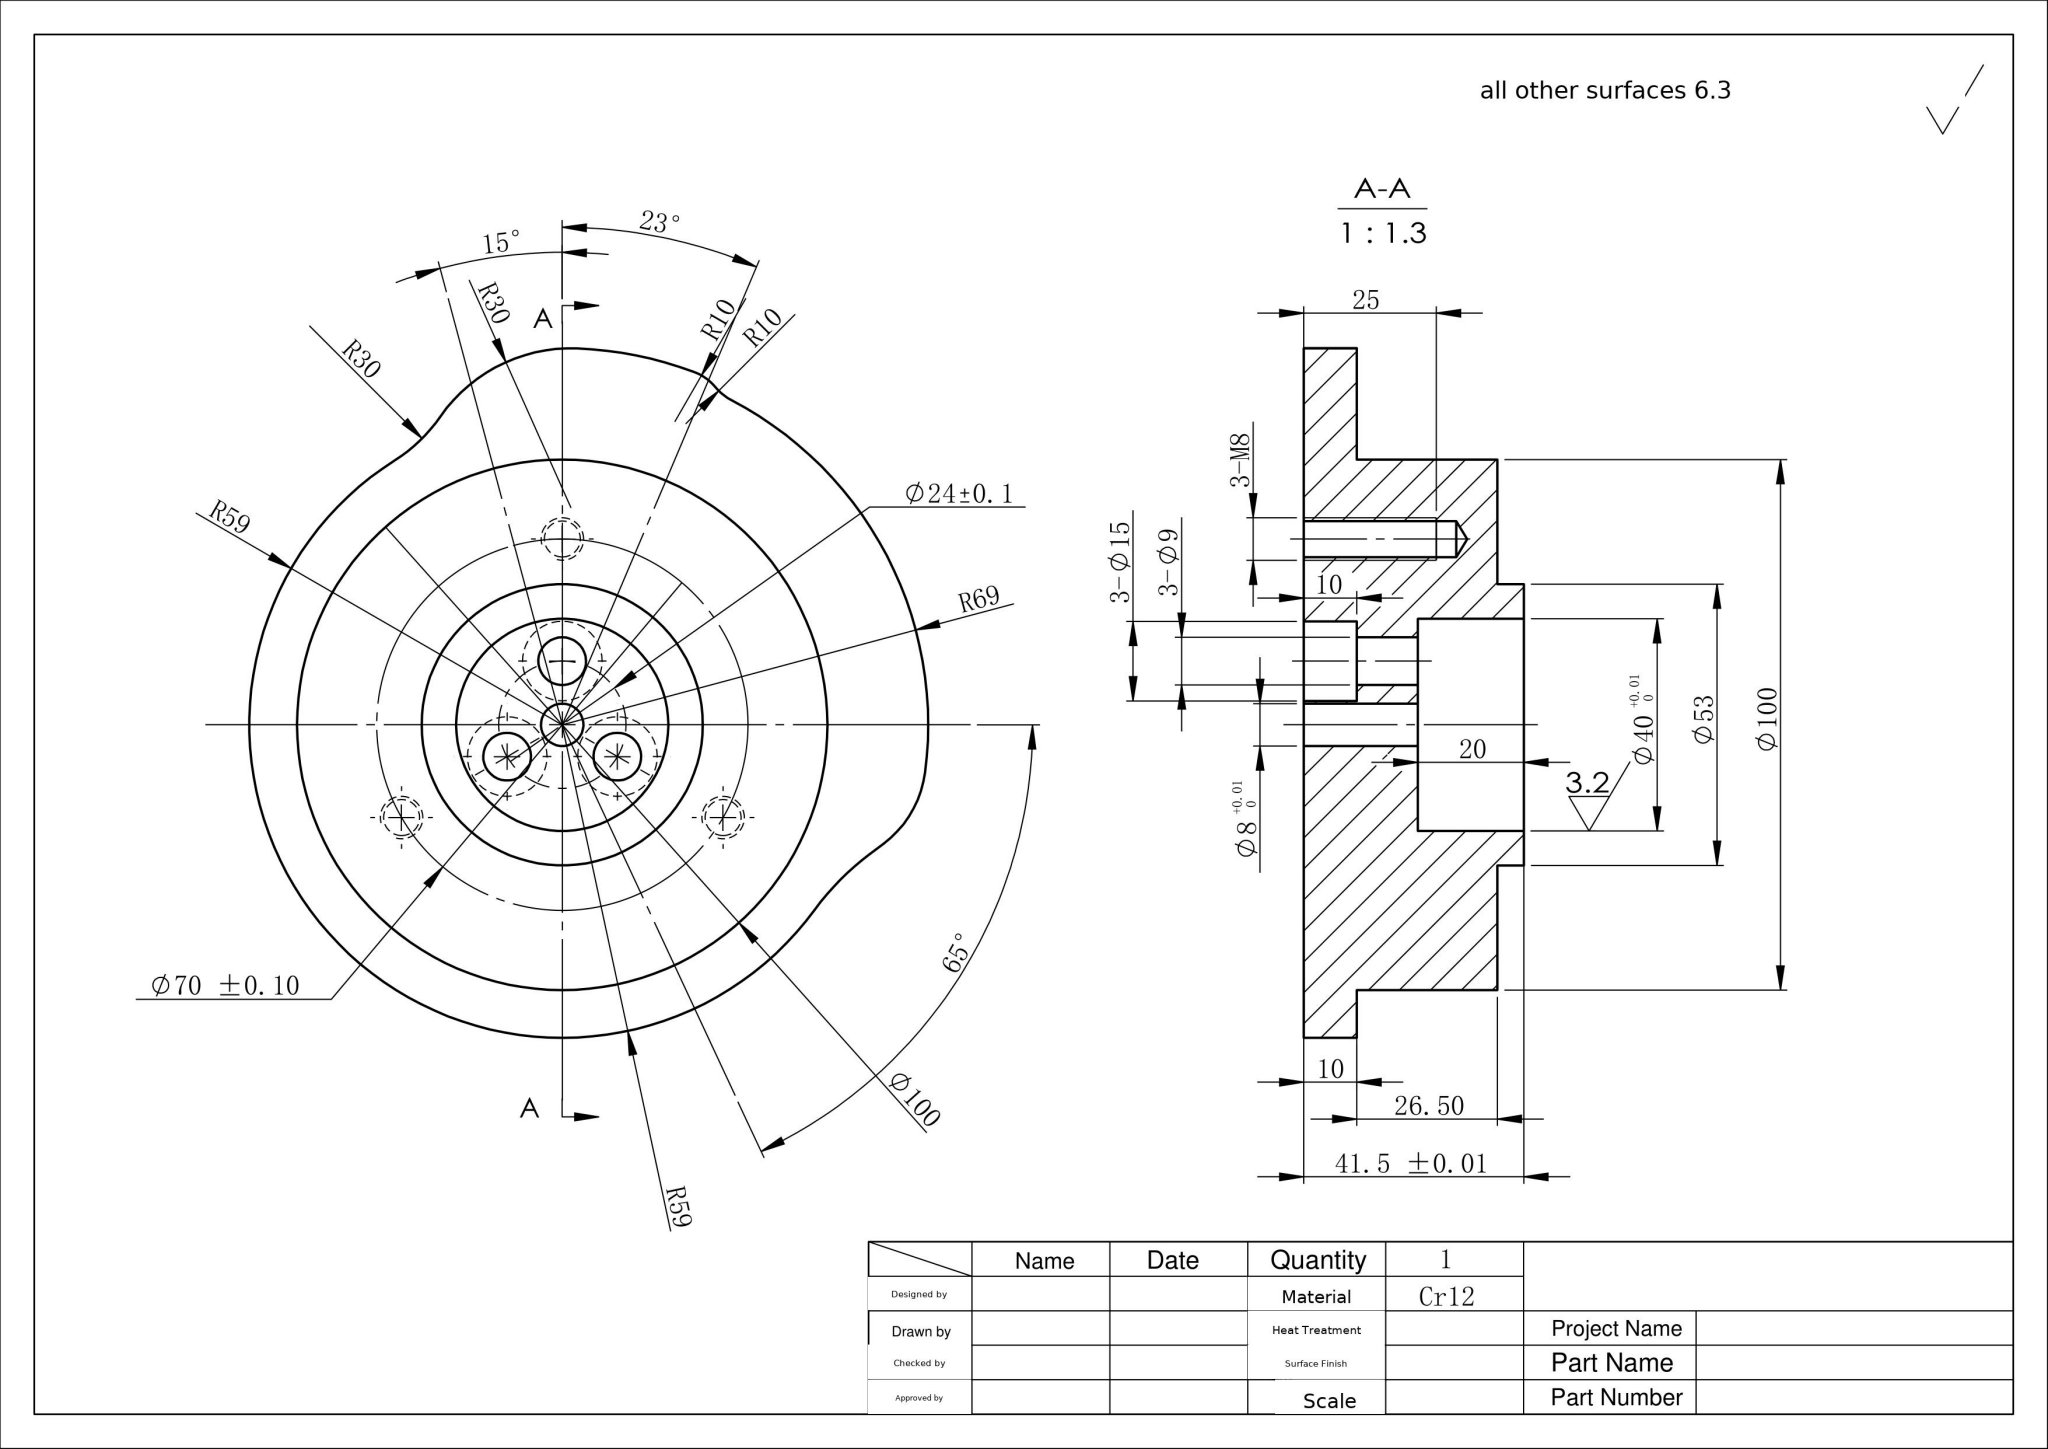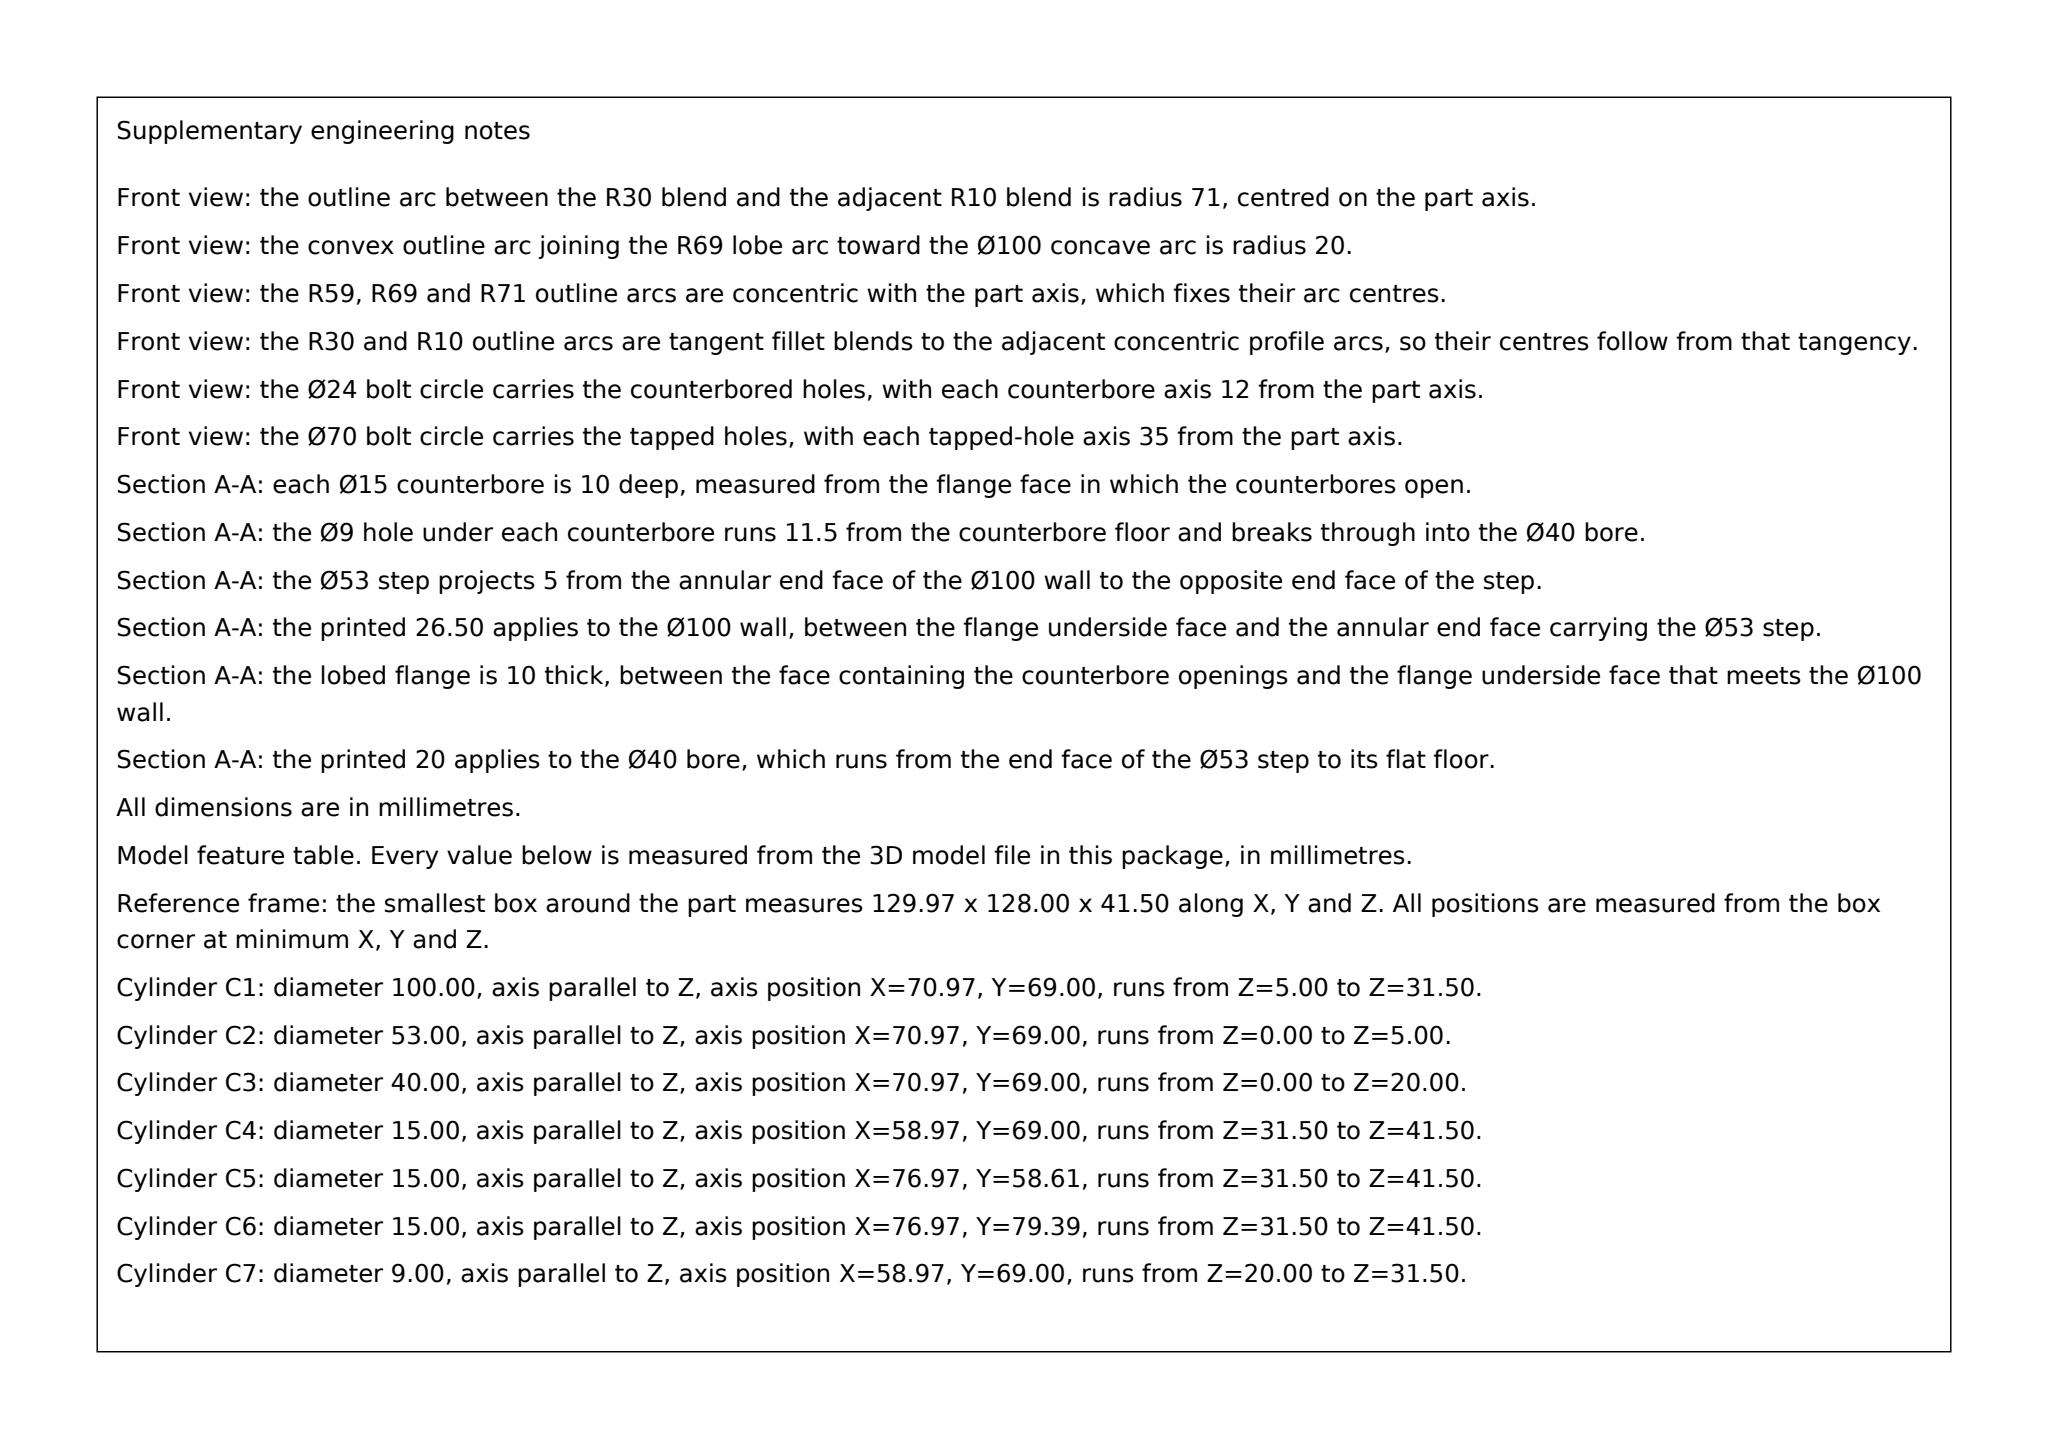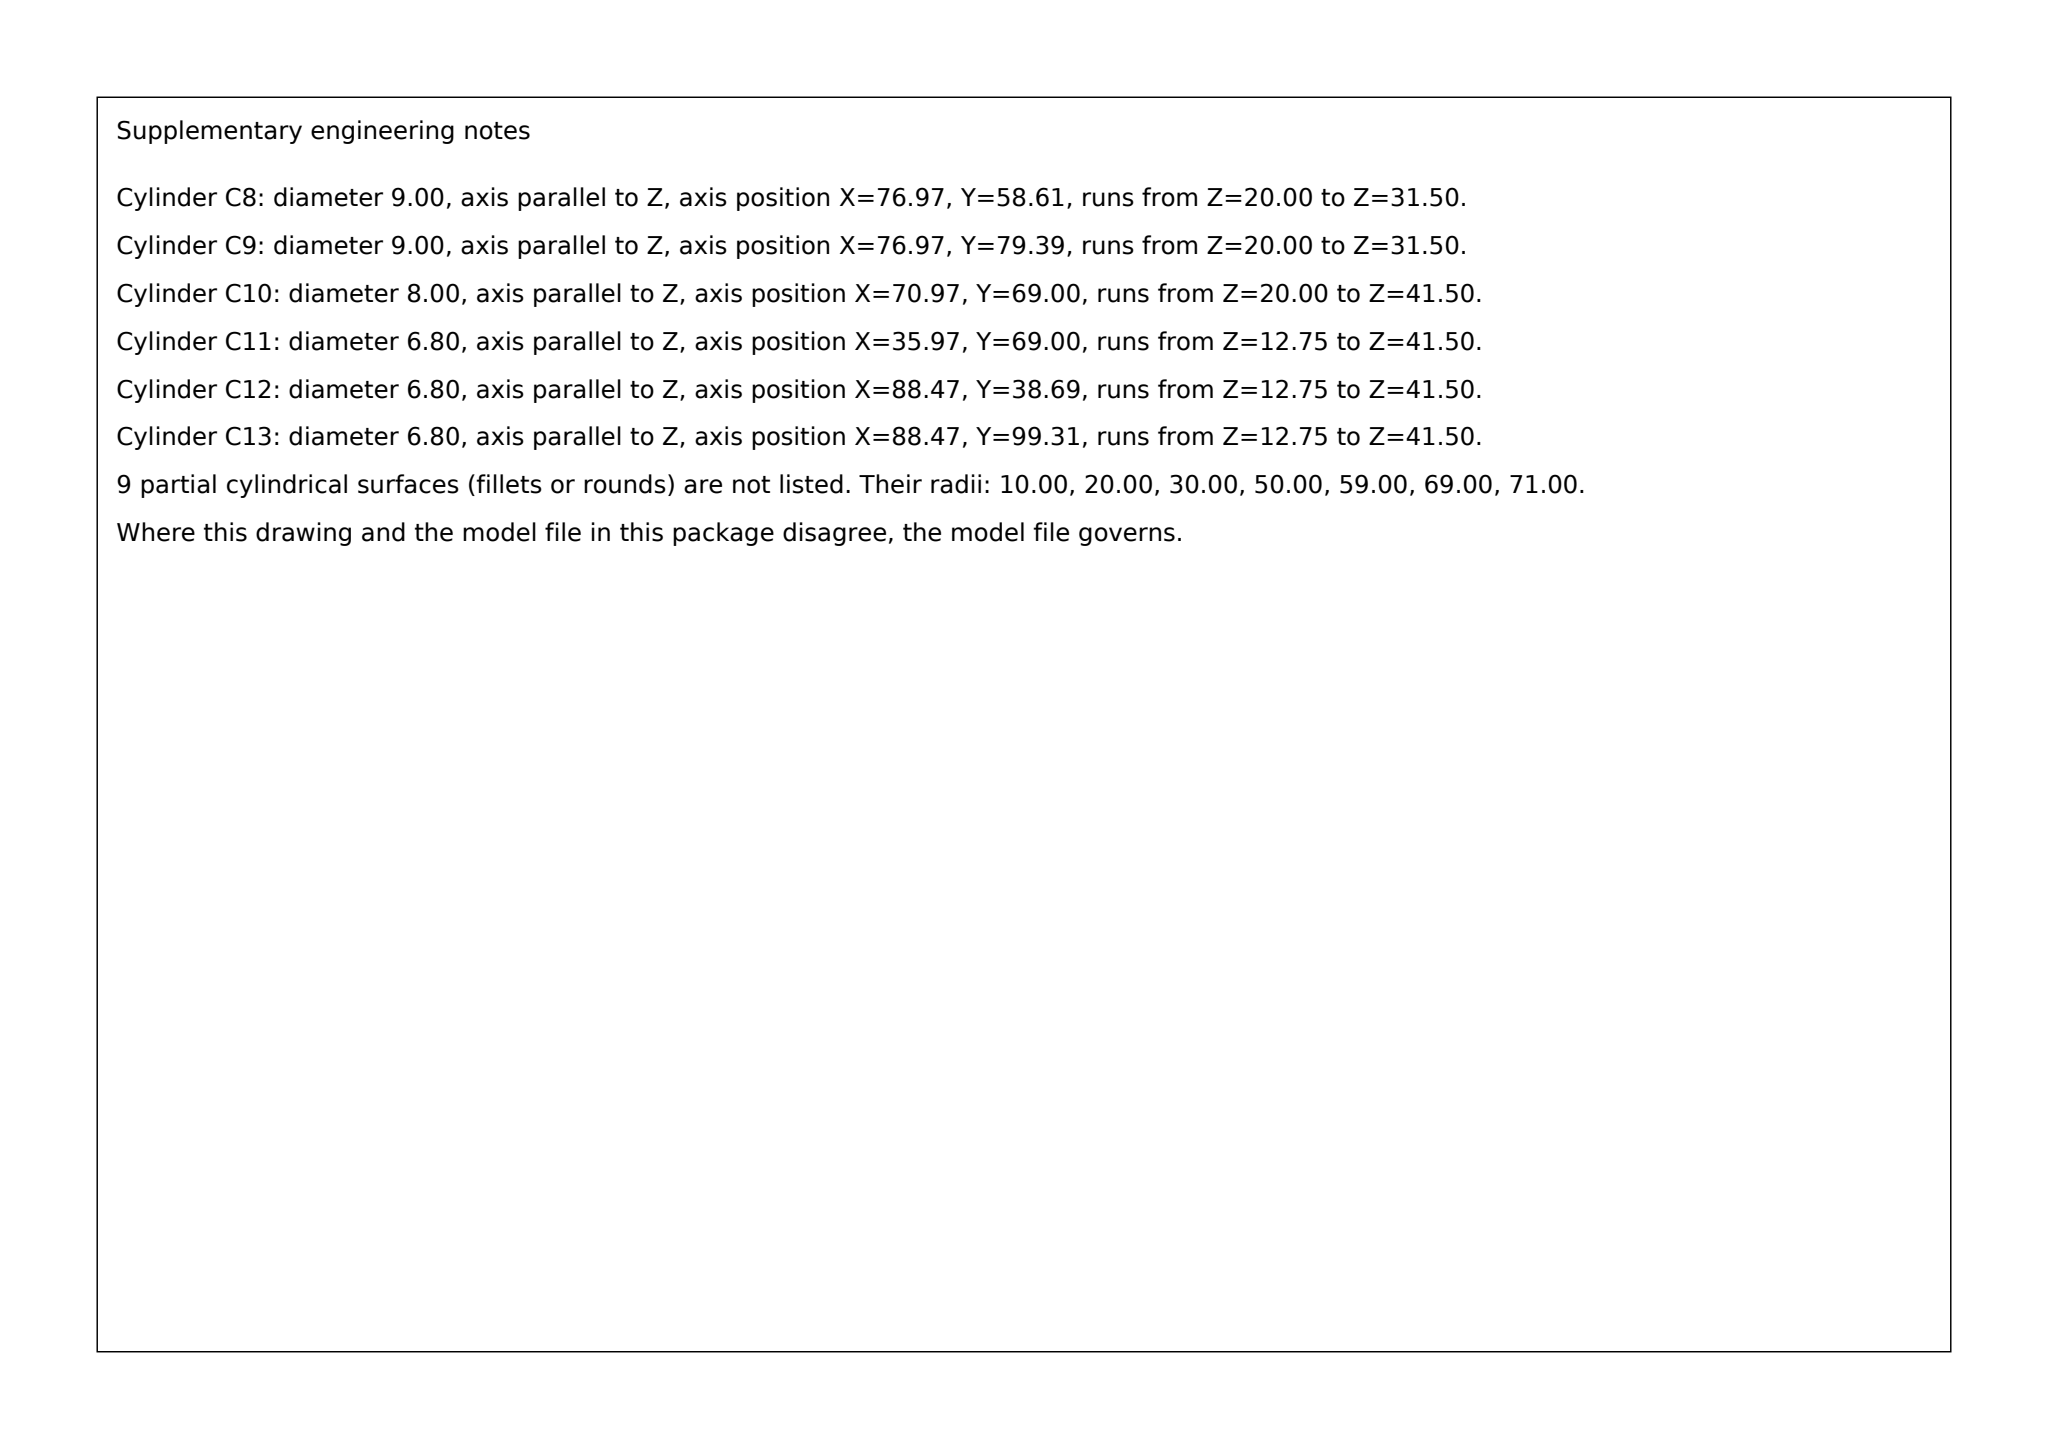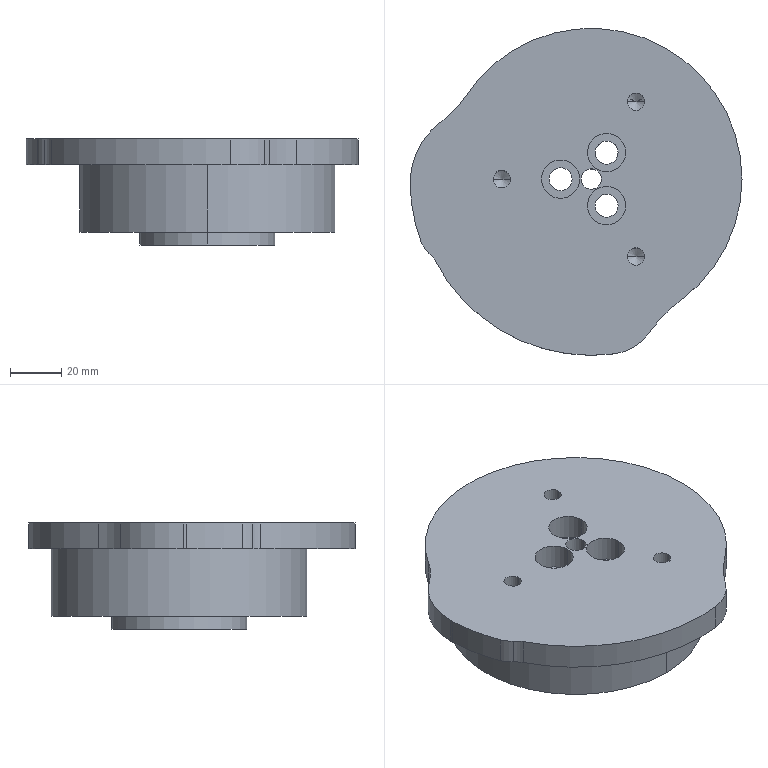Part | SolidWorks | mm | 1 solid | 52 faces | box 129.97 x 128 x 41.5 mm | volume 306852 mm3 | cylinder 37 | plane 9 | cone 6 | commonest cylinder face diameters 15 x6 6.8 x6 9 x6 60 x3 100 x3 40 x3 53 x2 8 x2
Drawing notes:
Ø8 +0.01/0 BLIND BORE DP 21.5 FROM LH FACE (A-A) | from the solid: cylinder dia 8.0 axis z at (70.97,69.0), length 21.5, blind (planes z=0..41.5)
3-M8 TAP DRILL Ø6.8 DP 28.75 FROM LH FACE, 118° PT | from the solid: 3 off cylinder dia 6.8 axis z, length 28.75, cones 118° incl on ref dia 6.8
3-Ø9 DP 11.5 FROM LH FACE (1.5 BELOW Ø15 CBORE DP 10) | from the solid: cylinders dia 9.0 length 11.5 coaxial with dia 15.0 length 10.0, 3 off
3-M8 EQ SP 120° ON Ø70 BC; ONE HOLE ON SECT A-A CL | from the solid: Ø6.8 tap drills at (35.97,69.0), (88.47,38.69), (88.47,99.31) vs part axis (70.97,69.0): R35 at 180°, -60°, +60° => Ø70 BC, 120° spacing, one on the vertical section axis
3-Ø9 W/ Ø15 C'BORE EQ SP 120° ON Ø24 BC; CLOCKED W/ M8 HOLES | from the solid: Ø9/Ø15 holes at (58.97,69.0), (76.97,58.61), (76.97,79.39) vs axis (70.97,69.0): R12 at 180°, -60°, +60° => Ø24 BC, 120° spacing, same angular clocking as the Ø70 M8 pattern